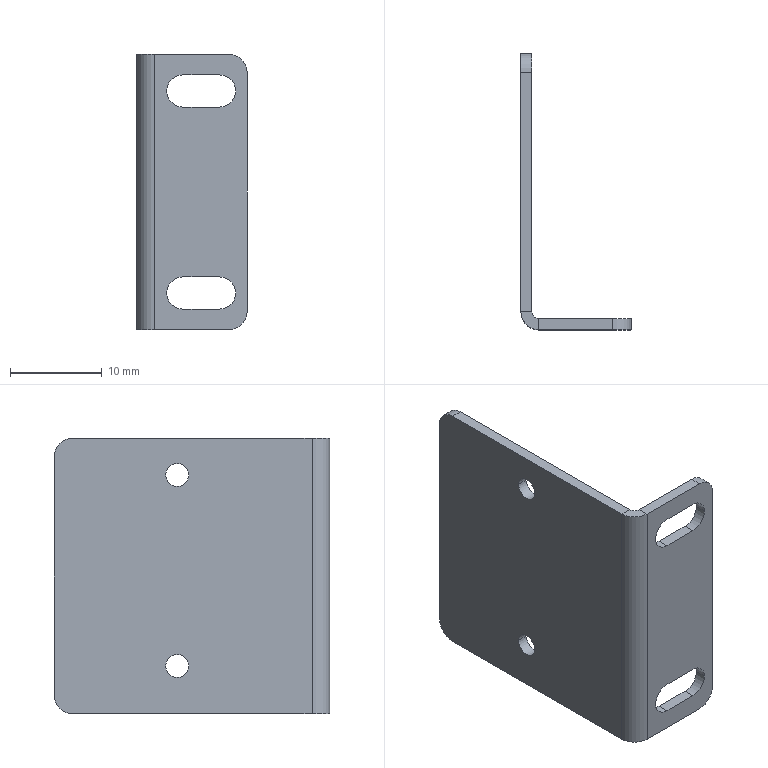Component | SolidWorks | SensorPlate7-1 | 1 solid | 32 faces | box 12 x 30 x 30 mm | volume 1376 mm3 | cylinder 16 | plane 16 | commonest cylinder face diameters 3.5 x6 2.5 x4 4 x4 3.873 x1 1.473 x1
STEP:
#1=COLOUR_RGB('',0.7922,0.8196,0.9333);
#2=FILL_AREA_STYLE_COLOUR('',#1);
#3=FILL_AREA_STYLE('',(#2));
#4=SURFACE_STYLE_FILL_AREA(#3);
#5=SURFACE_SIDE_STYLE('',(#4));
#6=SURFACE_STYLE_USAGE(.BOTH.,#5);
#7=PRESENTATION_STYLE_ASSIGNMENT((#6));
#8=CARTESIAN_POINT('',(-0.927,2.714,-3.325));
#9=VERTEX_POINT('',#8);
#10=CARTESIAN_POINT('',(-0.9958,2.714,-3.394));
#11=VERTEX_POINT('',#10);
#12=CARTESIAN_POINT('',(-0.9958,2.714,-3.325));
#13=DIRECTION('',(0.,1.,0.));
#14=DIRECTION('',(-1.,0.,0.));
#15=AXIS2_PLACEMENT_3D('',#12,#13,#14);
#16=CIRCLE('',#15,0.0689);
#17=EDGE_CURVE('',#9,#11,#16,.T.);
#18=ORIENTED_EDGE('',*,*,#17,.F.);
#19=CARTESIAN_POINT('',(-0.927,2.762,-3.325));
#20=VERTEX_POINT('',#19);
#21=CARTESIAN_POINT('',(-0.927,2.368,-3.325));
#22=DIRECTION('',(0.,1.,0.));
#23=VECTOR('',#22,39.37);
#24=LINE('',#21,#23);
#25=EDGE_CURVE('',#9,#20,#24,.T.);
#26=ORIENTED_EDGE('',*,*,#25,.T.);
#27=CARTESIAN_POINT('',(-0.9958,2.762,-3.394));
#28=VERTEX_POINT('',#27);
#29=CARTESIAN_POINT('',(-0.9958,2.762,-3.325));
#30=DIRECTION('',(-0.,-1.,-0.));
#31=DIRECTION('',(-1.,0.,0.));
#32=AXIS2_PLACEMENT_3D('',#29,#30,#31);
#33=CIRCLE('',#32,0.0689);
#34=EDGE_CURVE('',#28,#20,#33,.T.);
#35=ORIENTED_EDGE('',*,*,#34,.F.);
#36=CARTESIAN_POINT('',(-0.9958,2.368,-3.394));
#37=DIRECTION('',(0.,1.,0.));
#38=VECTOR('',#37,39.37);
#39=LINE('',#36,#38);
#40=EDGE_CURVE('',#11,#28,#39,.T.);
#41=ORIENTED_EDGE('',*,*,#40,.F.);
#42=EDGE_LOOP('',(#18,#26,#35,#41));
#43=FACE_OUTER_BOUND('',#42,.T.);
#44=CARTESIAN_POINT('',(-0.9958,2.368,-3.325));
#45=DIRECTION('',(0.,1.,0.));
#46=DIRECTION('',(1.,0.,0.));
#47=AXIS2_PLACEMENT_3D('',#44,#45,#46);
#48=CYLINDRICAL_SURFACE('',#47,0.0689);
#49=ADVANCED_FACE('',(#43),#48,.F.);
#50=CARTESIAN_POINT('',(-0.9958,2.714,-4.26));
#51=VERTEX_POINT('',#50);
#52=CARTESIAN_POINT('',(-0.927,2.714,-4.191));
#53=VERTEX_POINT('',#52);
#54=CARTESIAN_POINT('',(-0.9958,2.714,-4.191));
#55=DIRECTION('',(-0.,-1.,-0.));
#56=DIRECTION('',(-1.,0.,0.));
#57=AXIS2_PLACEMENT_3D('',#54,#55,#56);
#58=CIRCLE('',#57,0.0689);
#59=EDGE_CURVE('',#51,#53,#58,.T.);
#60=ORIENTED_EDGE('',*,*,#59,.T.);
#61=CARTESIAN_POINT('',(-0.927,2.762,-4.191));
#62=VERTEX_POINT('',#61);
#63=CARTESIAN_POINT('',(-0.927,2.368,-4.191));
#64=DIRECTION('',(0.,1.,0.));
#65=VECTOR('',#64,39.37);
#66=LINE('',#63,#65);
#67=EDGE_CURVE('',#53,#62,#66,.T.);
#68=ORIENTED_EDGE('',*,*,#67,.T.);
#69=CARTESIAN_POINT('',(-0.9958,2.762,-4.26));
#70=VERTEX_POINT('',#69);
#71=CARTESIAN_POINT('',(-0.9958,2.762,-4.191));
#72=DIRECTION('',(0.,1.,0.));
#73=DIRECTION('',(1.,0.,0.));
#74=AXIS2_PLACEMENT_3D('',#71,#72,#73);
#75=CIRCLE('',#74,0.0689);
#76=EDGE_CURVE('',#62,#70,#75,.T.);
#77=ORIENTED_EDGE('',*,*,#76,.T.);
#78=CARTESIAN_POINT('',(-0.9958,2.368,-4.26));
#79=DIRECTION('',(0.,1.,0.));
#80=VECTOR('',#79,39.37);
#81=LINE('',#78,#80);
#82=EDGE_CURVE('',#51,#70,#81,.T.);
#83=ORIENTED_EDGE('',*,*,#82,.F.);
#84=EDGE_LOOP('',(#60,#68,#77,#83));
#85=FACE_OUTER_BOUND('',#84,.T.);
#86=CARTESIAN_POINT('',(-0.9958,2.368,-4.191));
#87=DIRECTION('',(0.,1.,0.));
#88=DIRECTION('',(1.,0.,0.));
#89=AXIS2_PLACEMENT_3D('',#86,#87,#88);
#90=CYLINDRICAL_SURFACE('',#89,0.0689);
#91=ADVANCED_FACE('',(#85),#90,.F.);
#92=CARTESIAN_POINT('',(-1.303,3.417,-4.144));
#93=VERTEX_POINT('',#92);
#94=CARTESIAN_POINT('',(-1.303,3.319,-4.144));
#95=VERTEX_POINT('',#94);
#96=CARTESIAN_POINT('',(-1.303,3.368,-4.144));
#97=DIRECTION('',(1.,0.,-0.));
#98=DIRECTION('',(0.,-1.,0.));
#99=AXIS2_PLACEMENT_3D('',#96,#97,#98);
#100=CIRCLE('',#99,0.04921);
#101=EDGE_CURVE('',#93,#95,#100,.T.);
#102=ORIENTED_EDGE('',*,*,#101,.T.);
#103=CARTESIAN_POINT('',(-1.35,3.319,-4.144));
#104=VERTEX_POINT('',#103);
#105=CARTESIAN_POINT('',(-1.35,3.319,-4.144));
#106=DIRECTION('',(-1.,-0.,0.));
#107=VECTOR('',#106,39.37);
#108=LINE('',#105,#107);
#109=EDGE_CURVE('',#95,#104,#108,.T.);
#110=ORIENTED_EDGE('',*,*,#109,.T.);
#111=CARTESIAN_POINT('',(-1.35,3.417,-4.144));
#112=VERTEX_POINT('',#111);
#113=CARTESIAN_POINT('',(-1.35,3.368,-4.144));
#114=DIRECTION('',(-1.,-0.,0.));
#115=DIRECTION('',(0.,1.,0.));
#116=AXIS2_PLACEMENT_3D('',#113,#114,#115);
#117=CIRCLE('',#116,0.04921);
#118=EDGE_CURVE('',#104,#112,#117,.T.);
#119=ORIENTED_EDGE('',*,*,#118,.T.);
#120=CARTESIAN_POINT('',(-1.35,3.417,-4.144));
#121=DIRECTION('',(-1.,-0.,0.));
#122=VECTOR('',#121,39.37);
#123=LINE('',#120,#122);
#124=EDGE_CURVE('',#93,#112,#123,.T.);
#125=ORIENTED_EDGE('',*,*,#124,.F.);
#126=EDGE_LOOP('',(#102,#110,#119,#125));
#127=FACE_OUTER_BOUND('',#126,.T.);
#128=CARTESIAN_POINT('',(-1.35,3.368,-4.144));
#129=DIRECTION('',(-1.,-0.,0.));
#130=DIRECTION('',(0.,1.,0.));
#131=AXIS2_PLACEMENT_3D('',#128,#129,#130);
#132=CYLINDRICAL_SURFACE('',#131,0.04921);
#133=ADVANCED_FACE('',(#127),#132,.F.);
#134=CARTESIAN_POINT('',(-1.303,3.417,-3.325));
#135=VERTEX_POINT('',#134);
#136=CARTESIAN_POINT('',(-1.303,3.319,-3.325));
#137=VERTEX_POINT('',#136);
#138=CARTESIAN_POINT('',(-1.303,3.368,-3.325));
#139=DIRECTION('',(1.,0.,-0.));
#140=DIRECTION('',(0.,-1.,0.));
#141=AXIS2_PLACEMENT_3D('',#138,#139,#140);
#142=CIRCLE('',#141,0.04921);
#143=EDGE_CURVE('',#135,#137,#142,.T.);
#144=ORIENTED_EDGE('',*,*,#143,.T.);
#145=CARTESIAN_POINT('',(-1.35,3.319,-3.325));
#146=VERTEX_POINT('',#145);
#147=CARTESIAN_POINT('',(-1.35,3.319,-3.325));
#148=DIRECTION('',(-1.,-0.,0.));
#149=VECTOR('',#148,39.37);
#150=LINE('',#147,#149);
#151=EDGE_CURVE('',#137,#146,#150,.T.);
#152=ORIENTED_EDGE('',*,*,#151,.T.);
#153=CARTESIAN_POINT('',(-1.35,3.417,-3.325));
#154=VERTEX_POINT('',#153);
#155=CARTESIAN_POINT('',(-1.35,3.368,-3.325));
#156=DIRECTION('',(-1.,-0.,0.));
#157=DIRECTION('',(0.,1.,0.));
#158=AXIS2_PLACEMENT_3D('',#155,#156,#157);
#159=CIRCLE('',#158,0.04921);
#160=EDGE_CURVE('',#146,#154,#159,.T.);
#161=ORIENTED_EDGE('',*,*,#160,.T.);
#162=CARTESIAN_POINT('',(-1.35,3.417,-3.325));
#163=DIRECTION('',(-1.,-0.,0.));
#164=VECTOR('',#163,39.37);
#165=LINE('',#162,#164);
#166=EDGE_CURVE('',#135,#154,#165,.T.);
#167=ORIENTED_EDGE('',*,*,#166,.F.);
#168=EDGE_LOOP('',(#144,#152,#161,#167));
#169=FACE_OUTER_BOUND('',#168,.T.);
#170=CARTESIAN_POINT('',(-1.35,3.368,-3.325));
#171=DIRECTION('',(-1.,-0.,0.));
#172=DIRECTION('',(0.,1.,0.));
#173=AXIS2_PLACEMENT_3D('',#170,#171,#172);
#174=CYLINDRICAL_SURFACE('',#173,0.04921);
#175=ADVANCED_FACE('',(#169),#174,.F.);
#176=ORIENTED_EDGE('',*,*,#59,.F.);
#177=CARTESIAN_POINT('',(-1.153,2.714,-4.26));
#178=VERTEX_POINT('',#177);
#179=CARTESIAN_POINT('',(-1.303,2.714,-4.26));
#180=DIRECTION('',(1.,-0.,0.));
#181=VECTOR('',#180,39.37);
#182=LINE('',#179,#181);
#183=EDGE_CURVE('',#178,#51,#182,.T.);
#184=ORIENTED_EDGE('',*,*,#183,.F.);
#185=CARTESIAN_POINT('',(-1.153,2.714,-4.122));
#186=VERTEX_POINT('',#185);
#187=CARTESIAN_POINT('',(-1.153,2.714,-4.191));
#188=DIRECTION('',(-0.,-1.,-0.));
#189=DIRECTION('',(-1.,0.,0.));
#190=AXIS2_PLACEMENT_3D('',#187,#188,#189);
#191=CIRCLE('',#190,0.0689);
#192=EDGE_CURVE('',#186,#178,#191,.T.);
#193=ORIENTED_EDGE('',*,*,#192,.F.);
#194=CARTESIAN_POINT('',(-0.9958,2.714,-4.122));
#195=VERTEX_POINT('',#194);
#196=CARTESIAN_POINT('',(-1.303,2.714,-4.122));
#197=DIRECTION('',(1.,-0.,-0.));
#198=VECTOR('',#197,39.37);
#199=LINE('',#196,#198);
#200=EDGE_CURVE('',#186,#195,#199,.T.);
#201=ORIENTED_EDGE('',*,*,#200,.T.);
#202=CARTESIAN_POINT('',(-0.9958,2.714,-4.191));
#203=DIRECTION('',(-0.,-1.,-0.));
#204=DIRECTION('',(-1.,0.,0.));
#205=AXIS2_PLACEMENT_3D('',#202,#203,#204);
#206=CIRCLE('',#205,0.0689);
#207=EDGE_CURVE('',#53,#195,#206,.T.);
#208=ORIENTED_EDGE('',*,*,#207,.F.);
#209=EDGE_LOOP('',(#176,#184,#193,#201,#208));
#210=FACE_BOUND('',#209,.T.);
#211=CARTESIAN_POINT('',(-0.9565,2.714,-4.348));
#212=VERTEX_POINT('',#211);
#213=CARTESIAN_POINT('',(-1.274,2.714,-4.348));
#214=VERTEX_POINT('',#213);
#215=CARTESIAN_POINT('',(-1.303,2.714,-4.348));
#216=DIRECTION('',(-1.,0.,0.));
#217=VECTOR('',#216,39.37);
#218=LINE('',#215,#217);
#219=EDGE_CURVE('',#212,#214,#218,.T.);
#220=ORIENTED_EDGE('',*,*,#219,.F.);
#221=CARTESIAN_POINT('',(-0.8777,2.714,-4.27));
#222=VERTEX_POINT('',#221);
#223=CARTESIAN_POINT('',(-0.9565,2.714,-4.27));
#224=DIRECTION('',(-0.,-1.,-0.));
#225=DIRECTION('',(-1.,0.,0.));
#226=AXIS2_PLACEMENT_3D('',#223,#224,#225);
#227=CIRCLE('',#226,0.07874);
#228=EDGE_CURVE('',#212,#222,#227,.T.);
#229=ORIENTED_EDGE('',*,*,#228,.T.);
#230=CARTESIAN_POINT('',(-0.8777,2.714,-3.246));
#231=VERTEX_POINT('',#230);
#232=CARTESIAN_POINT('',(-0.8777,2.714,-4.348));
#233=DIRECTION('',(-0.,0.,-1.));
#234=VECTOR('',#233,39.37);
#235=LINE('',#232,#234);
#236=EDGE_CURVE('',#231,#222,#235,.T.);
#237=ORIENTED_EDGE('',*,*,#236,.F.);
#238=CARTESIAN_POINT('',(-0.9565,2.714,-3.167));
#239=VERTEX_POINT('',#238);
#240=CARTESIAN_POINT('',(-0.9565,2.714,-3.246));
#241=DIRECTION('',(-0.,-1.,-0.));
#242=DIRECTION('',(-1.,0.,0.));
#243=AXIS2_PLACEMENT_3D('',#240,#241,#242);
#244=CIRCLE('',#243,0.07874);
#245=EDGE_CURVE('',#231,#239,#244,.T.);
#246=ORIENTED_EDGE('',*,*,#245,.T.);
#247=CARTESIAN_POINT('',(-1.274,2.714,-3.167));
#248=VERTEX_POINT('',#247);
#249=CARTESIAN_POINT('',(-0.8777,2.714,-3.167));
#250=DIRECTION('',(1.,-0.,-0.));
#251=VECTOR('',#250,39.37);
#252=LINE('',#249,#251);
#253=EDGE_CURVE('',#248,#239,#252,.T.);
#254=ORIENTED_EDGE('',*,*,#253,.F.);
#255=CARTESIAN_POINT('',(-1.274,2.714,-3.561));
#256=DIRECTION('',(-0.,0.,-1.));
#257=VECTOR('',#256,39.37);
#258=LINE('',#255,#257);
#259=EDGE_CURVE('',#248,#214,#258,.T.);
#260=ORIENTED_EDGE('',*,*,#259,.T.);
#261=EDGE_LOOP('',(#220,#229,#237,#246,#254,#260));
#262=FACE_OUTER_BOUND('',#261,.T.);
#263=CARTESIAN_POINT('',(-1.153,2.714,-3.256));
#264=VERTEX_POINT('',#263);
#265=CARTESIAN_POINT('',(-0.9958,2.714,-3.256));
#266=VERTEX_POINT('',#265);
#267=CARTESIAN_POINT('',(-1.303,2.714,-3.256));
#268=DIRECTION('',(1.,-0.,-0.));
#269=VECTOR('',#268,39.37);
#270=LINE('',#267,#269);
#271=EDGE_CURVE('',#264,#266,#270,.T.);
#272=ORIENTED_EDGE('',*,*,#271,.T.);
#273=CARTESIAN_POINT('',(-0.9958,2.714,-3.325));
#274=DIRECTION('',(0.,1.,0.));
#275=DIRECTION('',(-1.,0.,0.));
#276=AXIS2_PLACEMENT_3D('',#273,#274,#275);
#277=CIRCLE('',#276,0.0689);
#278=EDGE_CURVE('',#266,#9,#277,.T.);
#279=ORIENTED_EDGE('',*,*,#278,.T.);
#280=ORIENTED_EDGE('',*,*,#17,.T.);
#281=CARTESIAN_POINT('',(-1.153,2.714,-3.394));
#282=VERTEX_POINT('',#281);
#283=CARTESIAN_POINT('',(-1.303,2.714,-3.394));
#284=DIRECTION('',(1.,-0.,-0.));
#285=VECTOR('',#284,39.37);
#286=LINE('',#283,#285);
#287=EDGE_CURVE('',#282,#11,#286,.T.);
#288=ORIENTED_EDGE('',*,*,#287,.F.);
#289=CARTESIAN_POINT('',(-1.153,2.714,-3.325));
#290=DIRECTION('',(0.,1.,0.));
#291=DIRECTION('',(-1.,0.,0.));
#292=AXIS2_PLACEMENT_3D('',#289,#290,#291);
#293=CIRCLE('',#292,0.0689);
#294=EDGE_CURVE('',#282,#264,#293,.T.);
#295=ORIENTED_EDGE('',*,*,#294,.T.);
#296=EDGE_LOOP('',(#272,#279,#280,#288,#295));
#297=FACE_BOUND('',#296,.T.);
#298=CARTESIAN_POINT('',(-1.303,2.714,-3.561));
#299=DIRECTION('',(-0.,-1.,-0.));
#300=DIRECTION('',(-1.,0.,0.));
#301=AXIS2_PLACEMENT_3D('',#298,#299,#300);
#302=PLANE('',#301);
#303=ADVANCED_FACE('',(#210,#262,#297),#302,.T.);
#304=CARTESIAN_POINT('',(-0.8777,2.762,-3.246));
#305=VERTEX_POINT('',#304);
#306=CARTESIAN_POINT('',(-0.8777,2.762,-4.27));
#307=VERTEX_POINT('',#306);
#308=CARTESIAN_POINT('',(-0.8777,2.762,-3.561));
#309=DIRECTION('',(-0.,0.,-1.));
#310=VECTOR('',#309,39.37);
#311=LINE('',#308,#310);
#312=EDGE_CURVE('',#305,#307,#311,.T.);
#313=ORIENTED_EDGE('',*,*,#312,.T.);
#314=CARTESIAN_POINT('',(-0.9565,2.762,-4.348));
#315=VERTEX_POINT('',#314);
#316=CARTESIAN_POINT('',(-0.9565,2.762,-4.27));
#317=DIRECTION('',(0.,1.,0.));
#318=DIRECTION('',(-1.,0.,0.));
#319=AXIS2_PLACEMENT_3D('',#316,#317,#318);
#320=CIRCLE('',#319,0.07874);
#321=EDGE_CURVE('',#307,#315,#320,.T.);
#322=ORIENTED_EDGE('',*,*,#321,.T.);
#323=CARTESIAN_POINT('',(-1.274,2.762,-4.348));
#324=VERTEX_POINT('',#323);
#325=CARTESIAN_POINT('',(-1.303,2.762,-4.348));
#326=DIRECTION('',(-1.,0.,0.));
#327=VECTOR('',#326,39.37);
#328=LINE('',#325,#327);
#329=EDGE_CURVE('',#315,#324,#328,.T.);
#330=ORIENTED_EDGE('',*,*,#329,.T.);
#331=CARTESIAN_POINT('',(-1.274,2.762,-3.167));
#332=VERTEX_POINT('',#331);
#333=CARTESIAN_POINT('',(-1.274,2.762,-3.167));
#334=DIRECTION('',(-0.,0.,-1.));
#335=VECTOR('',#334,39.37);
#336=LINE('',#333,#335);
#337=EDGE_CURVE('',#332,#324,#336,.T.);
#338=ORIENTED_EDGE('',*,*,#337,.F.);
#339=CARTESIAN_POINT('',(-0.9565,2.762,-3.167));
#340=VERTEX_POINT('',#339);
#341=CARTESIAN_POINT('',(-1.303,2.762,-3.167));
#342=DIRECTION('',(1.,-0.,-0.));
#343=VECTOR('',#342,39.37);
#344=LINE('',#341,#343);
#345=EDGE_CURVE('',#332,#340,#344,.T.);
#346=ORIENTED_EDGE('',*,*,#345,.T.);
#347=CARTESIAN_POINT('',(-0.9565,2.762,-3.246));
#348=DIRECTION('',(0.,1.,0.));
#349=DIRECTION('',(-1.,0.,0.));
#350=AXIS2_PLACEMENT_3D('',#347,#348,#349);
#351=CIRCLE('',#350,0.07874);
#352=EDGE_CURVE('',#340,#305,#351,.T.);
#353=ORIENTED_EDGE('',*,*,#352,.T.);
#354=EDGE_LOOP('',(#313,#322,#330,#338,#346,#353));
#355=FACE_OUTER_BOUND('',#354,.T.);
#356=CARTESIAN_POINT('',(-1.153,2.762,-4.26));
#357=VERTEX_POINT('',#356);
#358=CARTESIAN_POINT('',(-0.9958,2.762,-4.26));
#359=DIRECTION('',(-1.,0.,-0.));
#360=VECTOR('',#359,39.37);
#361=LINE('',#358,#360);
#362=EDGE_CURVE('',#70,#357,#361,.T.);
#363=ORIENTED_EDGE('',*,*,#362,.F.);
#364=ORIENTED_EDGE('',*,*,#76,.F.);
#365=CARTESIAN_POINT('',(-0.9958,2.762,-4.122));
#366=VERTEX_POINT('',#365);
#367=CARTESIAN_POINT('',(-0.9958,2.762,-4.191));
#368=DIRECTION('',(0.,1.,0.));
#369=DIRECTION('',(1.,0.,0.));
#370=AXIS2_PLACEMENT_3D('',#367,#368,#369);
#371=CIRCLE('',#370,0.0689);
#372=EDGE_CURVE('',#366,#62,#371,.T.);
#373=ORIENTED_EDGE('',*,*,#372,.F.);
#374=CARTESIAN_POINT('',(-1.153,2.762,-4.122));
#375=VERTEX_POINT('',#374);
#376=CARTESIAN_POINT('',(-0.9958,2.762,-4.122));
#377=DIRECTION('',(-1.,0.,0.));
#378=VECTOR('',#377,39.37);
#379=LINE('',#376,#378);
#380=EDGE_CURVE('',#366,#375,#379,.T.);
#381=ORIENTED_EDGE('',*,*,#380,.T.);
#382=CARTESIAN_POINT('',(-1.153,2.762,-4.191));
#383=DIRECTION('',(0.,1.,0.));
#384=DIRECTION('',(1.,0.,0.));
#385=AXIS2_PLACEMENT_3D('',#382,#383,#384);
#386=CIRCLE('',#385,0.0689);
#387=EDGE_CURVE('',#357,#375,#386,.T.);
#388=ORIENTED_EDGE('',*,*,#387,.F.);
#389=EDGE_LOOP('',(#363,#364,#373,#381,#388));
#390=FACE_BOUND('',#389,.T.);
#391=ORIENTED_EDGE('',*,*,#34,.T.);
#392=CARTESIAN_POINT('',(-0.9958,2.762,-3.256));
#393=VERTEX_POINT('',#392);
#394=CARTESIAN_POINT('',(-0.9958,2.762,-3.325));
#395=DIRECTION('',(-0.,-1.,-0.));
#396=DIRECTION('',(-1.,0.,0.));
#397=AXIS2_PLACEMENT_3D('',#394,#395,#396);
#398=CIRCLE('',#397,0.0689);
#399=EDGE_CURVE('',#20,#393,#398,.T.);
#400=ORIENTED_EDGE('',*,*,#399,.T.);
#401=CARTESIAN_POINT('',(-1.153,2.762,-3.256));
#402=VERTEX_POINT('',#401);
#403=CARTESIAN_POINT('',(-0.9958,2.762,-3.256));
#404=DIRECTION('',(-1.,0.,0.));
#405=VECTOR('',#404,39.37);
#406=LINE('',#403,#405);
#407=EDGE_CURVE('',#393,#402,#406,.T.);
#408=ORIENTED_EDGE('',*,*,#407,.T.);
#409=CARTESIAN_POINT('',(-1.153,2.762,-3.394));
#410=VERTEX_POINT('',#409);
#411=CARTESIAN_POINT('',(-1.153,2.762,-3.325));
#412=DIRECTION('',(-0.,-1.,-0.));
#413=DIRECTION('',(-1.,0.,0.));
#414=AXIS2_PLACEMENT_3D('',#411,#412,#413);
#415=CIRCLE('',#414,0.0689);
#416=EDGE_CURVE('',#402,#410,#415,.T.);
#417=ORIENTED_EDGE('',*,*,#416,.T.);
#418=CARTESIAN_POINT('',(-0.9958,2.762,-3.394));
#419=DIRECTION('',(-1.,0.,0.));
#420=VECTOR('',#419,39.37);
#421=LINE('',#418,#420);
#422=EDGE_CURVE('',#28,#410,#421,.T.);
#423=ORIENTED_EDGE('',*,*,#422,.F.);
#424=EDGE_LOOP('',(#391,#400,#408,#417,#423));
#425=FACE_BOUND('',#424,.T.);
#426=CARTESIAN_POINT('',(-1.303,2.762,-3.561));
#427=DIRECTION('',(-0.,-1.,-0.));
#428=DIRECTION('',(-1.,0.,0.));
#429=AXIS2_PLACEMENT_3D('',#426,#427,#428);
#430=PLANE('',#429);
#431=ADVANCED_FACE('',(#355,#390,#425),#430,.F.);
#432=CARTESIAN_POINT('',(-1.35,3.368,-4.144));
#433=DIRECTION('',(-1.,-0.,0.));
#434=DIRECTION('',(0.,1.,0.));
#435=AXIS2_PLACEMENT_3D('',#432,#433,#434);
#436=CIRCLE('',#435,0.04921);
#437=EDGE_CURVE('',#112,#104,#436,.T.);
#438=ORIENTED_EDGE('',*,*,#437,.F.);
#439=ORIENTED_EDGE('',*,*,#118,.F.);
#440=EDGE_LOOP('',(#438,#439));
#441=FACE_BOUND('',#440,.T.);
#442=CARTESIAN_POINT('',(-1.35,3.368,-3.325));
#443=DIRECTION('',(-1.,-0.,0.));
#444=DIRECTION('',(0.,1.,0.));
#445=AXIS2_PLACEMENT_3D('',#442,#443,#444);
#446=CIRCLE('',#445,0.04921);
#447=EDGE_CURVE('',#154,#146,#446,.T.);
#448=ORIENTED_EDGE('',*,*,#447,.F.);
#449=ORIENTED_EDGE('',*,*,#160,.F.);
#450=EDGE_LOOP('',(#448,#449));
#451=FACE_BOUND('',#450,.T.);
#452=CARTESIAN_POINT('',(-1.35,3.895,-3.246));
#453=VERTEX_POINT('',#452);
#454=CARTESIAN_POINT('',(-1.35,3.895,-4.27));
#455=VERTEX_POINT('',#454);
#456=CARTESIAN_POINT('',(-1.35,3.895,-3.167));
#457=DIRECTION('',(-0.,0.,-1.));
#458=VECTOR('',#457,39.37);
#459=LINE('',#456,#458);
#460=EDGE_CURVE('',#453,#455,#459,.T.);
#461=ORIENTED_EDGE('',*,*,#460,.T.);
#462=CARTESIAN_POINT('',(-1.35,3.817,-4.348));
#463=VERTEX_POINT('',#462);
#464=CARTESIAN_POINT('',(-1.35,3.817,-4.27));
#465=DIRECTION('',(-1.,-0.,0.));
#466=DIRECTION('',(0.,-1.,0.));
#467=AXIS2_PLACEMENT_3D('',#464,#465,#466);
#468=CIRCLE('',#467,0.07874);
#469=EDGE_CURVE('',#455,#463,#468,.T.);
#470=ORIENTED_EDGE('',*,*,#469,.T.);
#471=CARTESIAN_POINT('',(-1.35,2.791,-4.348));
#472=VERTEX_POINT('',#471);
#473=CARTESIAN_POINT('',(-1.35,2.714,-4.348));
#474=DIRECTION('',(-0.,1.,0.));
#475=VECTOR('',#474,39.37);
#476=LINE('',#473,#475);
#477=EDGE_CURVE('',#472,#463,#476,.T.);
#478=ORIENTED_EDGE('',*,*,#477,.F.);
#479=CARTESIAN_POINT('',(-1.35,2.791,-3.167));
#480=VERTEX_POINT('',#479);
#481=CARTESIAN_POINT('',(-1.35,2.791,-4.348));
#482=DIRECTION('',(0.,-0.,1.));
#483=VECTOR('',#482,39.37);
#484=LINE('',#481,#483);
#485=EDGE_CURVE('',#472,#480,#484,.T.);
#486=ORIENTED_EDGE('',*,*,#485,.T.);
#487=CARTESIAN_POINT('',(-1.35,3.817,-3.167));
#488=VERTEX_POINT('',#487);
#489=CARTESIAN_POINT('',(-1.35,2.714,-3.167));
#490=DIRECTION('',(-0.,1.,0.));
#491=VECTOR('',#490,39.37);
#492=LINE('',#489,#491);
#493=EDGE_CURVE('',#480,#488,#492,.T.);
#494=ORIENTED_EDGE('',*,*,#493,.T.);
#495=CARTESIAN_POINT('',(-1.35,3.817,-3.246));
#496=DIRECTION('',(-1.,-0.,0.));
#497=DIRECTION('',(0.,-1.,0.));
#498=AXIS2_PLACEMENT_3D('',#495,#496,#497);
#499=CIRCLE('',#498,0.07874);
#500=EDGE_CURVE('',#488,#453,#499,.T.);
#501=ORIENTED_EDGE('',*,*,#500,.T.);
#502=EDGE_LOOP('',(#461,#470,#478,#486,#494,#501));
#503=FACE_OUTER_BOUND('',#502,.T.);
#504=CARTESIAN_POINT('',(-1.35,2.714,-3.167));
#505=DIRECTION('',(1.,0.,-0.));
#506=DIRECTION('',(0.,-1.,-0.));
#507=AXIS2_PLACEMENT_3D('',#504,#505,#506);
#508=PLANE('',#507);
#509=ADVANCED_FACE('',(#441,#451,#503),#508,.F.);
#510=ORIENTED_EDGE('',*,*,#477,.T.);
#511=CARTESIAN_POINT('',(-1.303,3.817,-4.348));
#512=VERTEX_POINT('',#511);
#513=CARTESIAN_POINT('',(-1.303,3.817,-4.348));
#514=DIRECTION('',(1.,0.,-0.));
#515=VECTOR('',#514,39.37);
#516=LINE('',#513,#515);
#517=EDGE_CURVE('',#463,#512,#516,.T.);
#518=ORIENTED_EDGE('',*,*,#517,.T.);
#519=CARTESIAN_POINT('',(-1.303,2.791,-4.348));
#520=VERTEX_POINT('',#519);
#521=CARTESIAN_POINT('',(-1.303,2.714,-4.348));
#522=DIRECTION('',(-0.,1.,0.));
#523=VECTOR('',#522,39.37);
#524=LINE('',#521,#523);
#525=EDGE_CURVE('',#520,#512,#524,.T.);
#526=ORIENTED_EDGE('',*,*,#525,.F.);
#527=CARTESIAN_POINT('',(-1.303,2.791,-4.348));
#528=DIRECTION('',(-1.,-0.,0.));
#529=VECTOR('',#528,39.37);
#530=LINE('',#527,#529);
#531=EDGE_CURVE('',#520,#472,#530,.T.);
#532=ORIENTED_EDGE('',*,*,#531,.T.);
#533=EDGE_LOOP('',(#510,#518,#526,#532));
#534=FACE_OUTER_BOUND('',#533,.T.);
#535=CARTESIAN_POINT('',(-1.303,2.714,-4.348));
#536=DIRECTION('',(-0.,0.,-1.));
#537=DIRECTION('',(-0.,1.,0.));
#538=AXIS2_PLACEMENT_3D('',#535,#536,#537);
#539=PLANE('',#538);
#540=ADVANCED_FACE('',(#534),#539,.T.);
#541=ORIENTED_EDGE('',*,*,#101,.F.);
#542=CARTESIAN_POINT('',(-1.303,3.368,-4.144));
#543=DIRECTION('',(1.,0.,-0.));
#544=DIRECTION('',(0.,-1.,0.));
#545=AXIS2_PLACEMENT_3D('',#542,#543,#544);
#546=CIRCLE('',#545,0.04921);
#547=EDGE_CURVE('',#95,#93,#546,.T.);
#548=ORIENTED_EDGE('',*,*,#547,.F.);
#549=EDGE_LOOP('',(#541,#548));
#550=FACE_BOUND('',#549,.T.);
#551=ORIENTED_EDGE('',*,*,#143,.F.);
#552=CARTESIAN_POINT('',(-1.303,3.368,-3.325));
#553=DIRECTION('',(1.,0.,-0.));
#554=DIRECTION('',(0.,-1.,0.));
#555=AXIS2_PLACEMENT_3D('',#552,#553,#554);
#556=CIRCLE('',#555,0.04921);
#557=EDGE_CURVE('',#137,#135,#556,.T.);
#558=ORIENTED_EDGE('',*,*,#557,.F.);
#559=EDGE_LOOP('',(#551,#558));
#560=FACE_BOUND('',#559,.T.);
#561=ORIENTED_EDGE('',*,*,#525,.T.);
#562=CARTESIAN_POINT('',(-1.303,3.895,-4.27));
#563=VERTEX_POINT('',#562);
#564=CARTESIAN_POINT('',(-1.303,3.817,-4.27));
#565=DIRECTION('',(1.,0.,-0.));
#566=DIRECTION('',(0.,-1.,0.));
#567=AXIS2_PLACEMENT_3D('',#564,#565,#566);
#568=CIRCLE('',#567,0.07874);
#569=EDGE_CURVE('',#512,#563,#568,.T.);
#570=ORIENTED_EDGE('',*,*,#569,.T.);
#571=CARTESIAN_POINT('',(-1.303,3.895,-3.246));
#572=VERTEX_POINT('',#571);
#573=CARTESIAN_POINT('',(-1.303,3.895,-3.167));
#574=DIRECTION('',(-0.,0.,-1.));
#575=VECTOR('',#574,39.37);
#576=LINE('',#573,#575);
#577=EDGE_CURVE('',#572,#563,#576,.T.);
#578=ORIENTED_EDGE('',*,*,#577,.F.);
#579=CARTESIAN_POINT('',(-1.303,3.817,-3.167));
#580=VERTEX_POINT('',#579);
#581=CARTESIAN_POINT('',(-1.303,3.817,-3.246));
#582=DIRECTION('',(1.,0.,-0.));
#583=DIRECTION('',(0.,-1.,0.));
#584=AXIS2_PLACEMENT_3D('',#581,#582,#583);
#585=CIRCLE('',#584,0.07874);
#586=EDGE_CURVE('',#572,#580,#585,.T.);
#587=ORIENTED_EDGE('',*,*,#586,.T.);
#588=CARTESIAN_POINT('',(-1.303,2.791,-3.167));
#589=VERTEX_POINT('',#588);
#590=CARTESIAN_POINT('',(-1.303,2.714,-3.167));
#591=DIRECTION('',(-0.,1.,0.));
#592=VECTOR('',#591,39.37);
#593=LINE('',#590,#592);
#594=EDGE_CURVE('',#589,#580,#593,.T.);
#595=ORIENTED_EDGE('',*,*,#594,.F.);
#596=CARTESIAN_POINT('',(-1.303,2.791,-4.348));
#597=DIRECTION('',(0.,-0.,1.));
#598=VECTOR('',#597,39.37);
#599=LINE('',#596,#598);
#600=EDGE_CURVE('',#520,#589,#599,.T.);
#601=ORIENTED_EDGE('',*,*,#600,.F.);
#602=EDGE_LOOP('',(#561,#570,#578,#587,#595,#601));
#603=FACE_OUTER_BOUND('',#602,.T.);
#604=CARTESIAN_POINT('',(-1.303,2.714,-3.167));
#605=DIRECTION('',(1.,0.,-0.));
#606=DIRECTION('',(0.,-1.,-0.));
#607=AXIS2_PLACEMENT_3D('',#604,#605,#606);
#608=PLANE('',#607);
#609=ADVANCED_FACE('',(#550,#560,#603),#608,.T.);
#610=ORIENTED_EDGE('',*,*,#594,.T.);
#611=CARTESIAN_POINT('',(-1.35,3.817,-3.167));
#612=DIRECTION('',(-1.,-0.,0.));
#613=VECTOR('',#612,39.37);
#614=LINE('',#611,#613);
#615=EDGE_CURVE('',#580,#488,#614,.T.);
#616=ORIENTED_EDGE('',*,*,#615,.T.);
#617=ORIENTED_EDGE('',*,*,#493,.F.);
#618=CARTESIAN_POINT('',(-1.303,2.791,-3.167));
#619=DIRECTION('',(-1.,-0.,0.));
#620=VECTOR('',#619,39.37);
#621=LINE('',#618,#620);
#622=EDGE_CURVE('',#589,#480,#621,.T.);
#623=ORIENTED_EDGE('',*,*,#622,.F.);
#624=EDGE_LOOP('',(#610,#616,#617,#623));
#625=FACE_OUTER_BOUND('',#624,.T.);
#626=CARTESIAN_POINT('',(-1.35,2.714,-3.167));
#627=DIRECTION('',(0.,-0.,1.));
#628=DIRECTION('',(0.,-1.,-0.));
#629=AXIS2_PLACEMENT_3D('',#626,#627,#628);
#630=PLANE('',#629);
#631=ADVANCED_FACE('',(#625),#630,.T.);
#632=ORIENTED_EDGE('',*,*,#577,.T.);
#633=CARTESIAN_POINT('',(-1.303,3.895,-4.27));
#634=DIRECTION('',(-1.,-0.,0.));
#635=VECTOR('',#634,39.37);
#636=LINE('',#633,#635);
#637=EDGE_CURVE('',#563,#455,#636,.T.);
#638=ORIENTED_EDGE('',*,*,#637,.T.);
#639=ORIENTED_EDGE('',*,*,#460,.F.);
#640=CARTESIAN_POINT('',(-1.303,3.895,-3.246));
#641=DIRECTION('',(1.,0.,-0.));
#642=VECTOR('',#641,39.37);
#643=LINE('',#640,#642);
#644=EDGE_CURVE('',#453,#572,#643,.T.);
#645=ORIENTED_EDGE('',*,*,#644,.T.);
#646=EDGE_LOOP('',(#632,#638,#639,#645));
#647=FACE_OUTER_BOUND('',#646,.T.);
#648=CARTESIAN_POINT('',(-1.303,3.895,-3.561));
#649=DIRECTION('',(-0.,1.,0.));
#650=DIRECTION('',(0.,-0.,1.));
#651=AXIS2_PLACEMENT_3D('',#648,#649,#650);
#652=PLANE('',#651);
#653=ADVANCED_FACE('',(#647),#652,.T.);
#654=CARTESIAN_POINT('',(-1.274,2.714,-3.167));
#655=DIRECTION('',(0.,-1.,-0.));
#656=VECTOR('',#655,39.37);
#657=LINE('',#654,#656);
#658=EDGE_CURVE('',#332,#248,#657,.T.);
#659=ORIENTED_EDGE('',*,*,#658,.F.);
#660=CARTESIAN_POINT('',(-1.274,2.791,-3.167));
#661=DIRECTION('',(0.,-0.,1.));
#662=DIRECTION('',(0.,1.,0.));
#663=AXIS2_PLACEMENT_3D('',#660,#661,#662);
#664=CIRCLE('',#663,0.029);
#665=EDGE_CURVE('',#589,#332,#664,.T.);
#666=ORIENTED_EDGE('',*,*,#665,.F.);
#667=ORIENTED_EDGE('',*,*,#622,.T.);
#668=CARTESIAN_POINT('',(-1.274,2.791,-3.167));
#669=DIRECTION('',(0.,-0.,1.));
#670=DIRECTION('',(-0.,1.,0.));
#671=AXIS2_PLACEMENT_3D('',#668,#669,#670);
#672=CIRCLE('',#671,0.07624);
#673=EDGE_CURVE('',#480,#248,#672,.T.);
#674=ORIENTED_EDGE('',*,*,#673,.T.);
#675=EDGE_LOOP('',(#659,#666,#667,#674));
#676=FACE_OUTER_BOUND('',#675,.T.);
#677=CARTESIAN_POINT('',(-1.274,2.791,-3.167));
#678=DIRECTION('',(0.,-0.,1.));
#679=DIRECTION('',(0.,-1.,-0.));
#680=AXIS2_PLACEMENT_3D('',#677,#678,#679);
#681=PLANE('',#680);
#682=ADVANCED_FACE('',(#676),#681,.T.);
#683=CARTESIAN_POINT('',(-1.274,2.791,-4.348));
#684=DIRECTION('',(-0.,0.,-1.));
#685=DIRECTION('',(0.,1.,0.));
#686=AXIS2_PLACEMENT_3D('',#683,#684,#685);
#687=CIRCLE('',#686,0.029);
#688=EDGE_CURVE('',#324,#520,#687,.T.);
#689=ORIENTED_EDGE('',*,*,#688,.F.);
#690=CARTESIAN_POINT('',(-1.274,2.762,-4.348));
#691=DIRECTION('',(0.,-1.,-0.));
#692=VECTOR('',#691,39.37);
#693=LINE('',#690,#692);
#694=EDGE_CURVE('',#324,#214,#693,.T.);
#695=ORIENTED_EDGE('',*,*,#694,.T.);
#696=CARTESIAN_POINT('',(-1.274,2.791,-4.348));
#697=DIRECTION('',(-0.,0.,-1.));
#698=DIRECTION('',(-0.,1.,0.));
#699=AXIS2_PLACEMENT_3D('',#696,#697,#698);
#700=CIRCLE('',#699,0.07624);
#701=EDGE_CURVE('',#214,#472,#700,.T.);
#702=ORIENTED_EDGE('',*,*,#701,.T.);
#703=ORIENTED_EDGE('',*,*,#531,.F.);
#704=EDGE_LOOP('',(#689,#695,#702,#703));
#705=FACE_OUTER_BOUND('',#704,.T.);
#706=CARTESIAN_POINT('',(-1.274,2.791,-4.348));
#707=DIRECTION('',(0.,-0.,1.));
#708=DIRECTION('',(0.,-1.,-0.));
#709=AXIS2_PLACEMENT_3D('',#706,#707,#708);
#710=PLANE('',#709);
#711=ADVANCED_FACE('',(#705),#710,.F.);
#712=ORIENTED_EDGE('',*,*,#485,.F.);
#713=ORIENTED_EDGE('',*,*,#701,.F.);
#714=ORIENTED_EDGE('',*,*,#259,.F.);
#715=ORIENTED_EDGE('',*,*,#673,.F.);
#716=EDGE_LOOP('',(#712,#713,#714,#715));
#717=FACE_OUTER_BOUND('',#716,.T.);
#718=CARTESIAN_POINT('',(-1.274,2.791,-4.348));
#719=DIRECTION('',(-0.,0.,-1.));
#720=DIRECTION('',(0.,-1.,0.));
#721=AXIS2_PLACEMENT_3D('',#718,#719,#720);
#722=CYLINDRICAL_SURFACE('',#721,0.07624);
#723=ADVANCED_FACE('',(#717),#722,.T.);
#724=ORIENTED_EDGE('',*,*,#600,.T.);
#725=ORIENTED_EDGE('',*,*,#665,.T.);
#726=ORIENTED_EDGE('',*,*,#337,.T.);
#727=ORIENTED_EDGE('',*,*,#688,.T.);
#728=EDGE_LOOP('',(#724,#725,#726,#727));
#729=FACE_OUTER_BOUND('',#728,.T.);
#730=CARTESIAN_POINT('',(-1.274,2.791,-4.348));
#731=DIRECTION('',(-0.,0.,-1.));
#732=DIRECTION('',(0.,-1.,0.));
#733=AXIS2_PLACEMENT_3D('',#730,#731,#732);
#734=CYLINDRICAL_SURFACE('',#733,0.029);
#735=ADVANCED_FACE('',(#729),#734,.F.);
#736=ORIENTED_EDGE('',*,*,#329,.F.);
#737=CARTESIAN_POINT('',(-0.9565,2.714,-4.348));
#738=DIRECTION('',(-0.,-1.,-0.));
#739=VECTOR('',#738,39.37);
#740=LINE('',#737,#739);
#741=EDGE_CURVE('',#315,#212,#740,.T.);
#742=ORIENTED_EDGE('',*,*,#741,.T.);
#743=ORIENTED_EDGE('',*,*,#219,.T.);
#744=ORIENTED_EDGE('',*,*,#694,.F.);
#745=EDGE_LOOP('',(#736,#742,#743,#744));
#746=FACE_OUTER_BOUND('',#745,.T.);
#747=CARTESIAN_POINT('',(-1.303,2.714,-4.348));
#748=DIRECTION('',(-0.,0.,-1.));
#749=DIRECTION('',(-0.,1.,0.));
#750=AXIS2_PLACEMENT_3D('',#747,#748,#749);
#751=PLANE('',#750);
#752=ADVANCED_FACE('',(#746),#751,.T.);
#753=ORIENTED_EDGE('',*,*,#253,.T.);
#754=CARTESIAN_POINT('',(-0.9565,2.714,-3.167));
#755=DIRECTION('',(0.,1.,0.));
#756=VECTOR('',#755,39.37);
#757=LINE('',#754,#756);
#758=EDGE_CURVE('',#239,#340,#757,.T.);
#759=ORIENTED_EDGE('',*,*,#758,.T.);
#760=ORIENTED_EDGE('',*,*,#345,.F.);
#761=ORIENTED_EDGE('',*,*,#658,.T.);
#762=EDGE_LOOP('',(#753,#759,#760,#761));
#763=FACE_OUTER_BOUND('',#762,.T.);
#764=CARTESIAN_POINT('',(-0.8777,2.714,-3.167));
#765=DIRECTION('',(0.,-0.,1.));
#766=DIRECTION('',(0.,-1.,-0.));
#767=AXIS2_PLACEMENT_3D('',#764,#765,#766);
#768=PLANE('',#767);
#769=ADVANCED_FACE('',(#763),#768,.T.);
#770=ORIENTED_EDGE('',*,*,#236,.T.);
#771=CARTESIAN_POINT('',(-0.8777,2.714,-4.27));
#772=DIRECTION('',(0.,1.,0.));
#773=VECTOR('',#772,39.37);
#774=LINE('',#771,#773);
#775=EDGE_CURVE('',#222,#307,#774,.T.);
#776=ORIENTED_EDGE('',*,*,#775,.T.);
#777=ORIENTED_EDGE('',*,*,#312,.F.);
#778=CARTESIAN_POINT('',(-0.8777,2.714,-3.246));
#779=DIRECTION('',(-0.,-1.,-0.));
#780=VECTOR('',#779,39.37);
#781=LINE('',#778,#780);
#782=EDGE_CURVE('',#305,#231,#781,.T.);
#783=ORIENTED_EDGE('',*,*,#782,.T.);
#784=EDGE_LOOP('',(#770,#776,#777,#783));
#785=FACE_OUTER_BOUND('',#784,.T.);
#786=CARTESIAN_POINT('',(-0.8777,2.714,-4.348));
#787=DIRECTION('',(1.,-0.,-0.));
#788=DIRECTION('',(-0.,-1.,-0.));
#789=AXIS2_PLACEMENT_3D('',#786,#787,#788);
#790=PLANE('',#789);
#791=ADVANCED_FACE('',(#785),#790,.T.);
#792=ORIENTED_EDGE('',*,*,#228,.F.);
#793=ORIENTED_EDGE('',*,*,#741,.F.);
#794=ORIENTED_EDGE('',*,*,#321,.F.);
#795=ORIENTED_EDGE('',*,*,#775,.F.);
#796=EDGE_LOOP('',(#792,#793,#794,#795));
#797=FACE_OUTER_BOUND('',#796,.T.);
#798=CARTESIAN_POINT('',(-0.9565,2.714,-4.27));
#799=DIRECTION('',(0.,1.,0.));
#800=DIRECTION('',(1.,0.,0.));
#801=AXIS2_PLACEMENT_3D('',#798,#799,#800);
#802=CYLINDRICAL_SURFACE('',#801,0.07874);
#803=ADVANCED_FACE('',(#797),#802,.T.);
#804=ORIENTED_EDGE('',*,*,#245,.F.);
#805=ORIENTED_EDGE('',*,*,#782,.F.);
#806=ORIENTED_EDGE('',*,*,#352,.F.);
#807=ORIENTED_EDGE('',*,*,#758,.F.);
#808=EDGE_LOOP('',(#804,#805,#806,#807));
#809=FACE_OUTER_BOUND('',#808,.T.);
#810=CARTESIAN_POINT('',(-0.9565,2.714,-3.246));
#811=DIRECTION('',(0.,1.,0.));
#812=DIRECTION('',(1.,0.,0.));
#813=AXIS2_PLACEMENT_3D('',#810,#811,#812);
#814=CYLINDRICAL_SURFACE('',#813,0.07874);
#815=ADVANCED_FACE('',(#809),#814,.T.);
#816=ORIENTED_EDGE('',*,*,#569,.F.);
#817=ORIENTED_EDGE('',*,*,#517,.F.);
#818=ORIENTED_EDGE('',*,*,#469,.F.);
#819=ORIENTED_EDGE('',*,*,#637,.F.);
#820=EDGE_LOOP('',(#816,#817,#818,#819));
#821=FACE_OUTER_BOUND('',#820,.T.);
#822=CARTESIAN_POINT('',(-1.303,3.817,-4.27));
#823=DIRECTION('',(-1.,-0.,0.));
#824=DIRECTION('',(-0.,1.,0.));
#825=AXIS2_PLACEMENT_3D('',#822,#823,#824);
#826=CYLINDRICAL_SURFACE('',#825,0.07874);
#827=ADVANCED_FACE('',(#821),#826,.T.);
#828=ORIENTED_EDGE('',*,*,#500,.F.);
#829=ORIENTED_EDGE('',*,*,#615,.F.);
#830=ORIENTED_EDGE('',*,*,#586,.F.);
#831=ORIENTED_EDGE('',*,*,#644,.F.);
#832=EDGE_LOOP('',(#828,#829,#830,#831));
#833=FACE_OUTER_BOUND('',#832,.T.);
#834=CARTESIAN_POINT('',(-1.303,3.817,-3.246));
#835=DIRECTION('',(1.,0.,-0.));
#836=DIRECTION('',(0.,-1.,0.));
#837=AXIS2_PLACEMENT_3D('',#834,#835,#836);
#838=CYLINDRICAL_SURFACE('',#837,0.07874);
#839=ADVANCED_FACE('',(#833),#838,.T.);
#840=ORIENTED_EDGE('',*,*,#151,.F.);
#841=ORIENTED_EDGE('',*,*,#557,.T.);
#842=ORIENTED_EDGE('',*,*,#166,.T.);
#843=ORIENTED_EDGE('',*,*,#447,.T.);
#844=EDGE_LOOP('',(#840,#841,#842,#843));
#845=FACE_OUTER_BOUND('',#844,.T.);
#846=CARTESIAN_POINT('',(-1.35,3.368,-3.325));
#847=DIRECTION('',(-1.,-0.,0.));
#848=DIRECTION('',(0.,1.,0.));
#849=AXIS2_PLACEMENT_3D('',#846,#847,#848);
#850=CYLINDRICAL_SURFACE('',#849,0.04921);
#851=ADVANCED_FACE('',(#845),#850,.F.);
#852=ORIENTED_EDGE('',*,*,#109,.F.);
#853=ORIENTED_EDGE('',*,*,#547,.T.);
#854=ORIENTED_EDGE('',*,*,#124,.T.);
#855=ORIENTED_EDGE('',*,*,#437,.T.);
#856=EDGE_LOOP('',(#852,#853,#854,#855));
#857=FACE_OUTER_BOUND('',#856,.T.);
#858=CARTESIAN_POINT('',(-1.35,3.368,-4.144));
#859=DIRECTION('',(-1.,-0.,0.));
#860=DIRECTION('',(0.,1.,0.));
#861=AXIS2_PLACEMENT_3D('',#858,#859,#860);
#862=CYLINDRICAL_SURFACE('',#861,0.04921);
#863=ADVANCED_FACE('',(#857),#862,.F.);
#864=ORIENTED_EDGE('',*,*,#67,.F.);
#865=ORIENTED_EDGE('',*,*,#207,.T.);
#866=CARTESIAN_POINT('',(-0.9958,2.368,-4.122));
#867=DIRECTION('',(0.,1.,0.));
#868=VECTOR('',#867,39.37);
#869=LINE('',#866,#868);
#870=EDGE_CURVE('',#195,#366,#869,.T.);
#871=ORIENTED_EDGE('',*,*,#870,.T.);
#872=ORIENTED_EDGE('',*,*,#372,.T.);
#873=EDGE_LOOP('',(#864,#865,#871,#872));
#874=FACE_OUTER_BOUND('',#873,.T.);
#875=CARTESIAN_POINT('',(-0.9958,2.368,-4.191));
#876=DIRECTION('',(0.,1.,0.));
#877=DIRECTION('',(1.,0.,0.));
#878=AXIS2_PLACEMENT_3D('',#875,#876,#877);
#879=CYLINDRICAL_SURFACE('',#878,0.0689);
#880=ADVANCED_FACE('',(#874),#879,.F.);
#881=CARTESIAN_POINT('',(-1.153,2.368,-4.122));
#882=DIRECTION('',(0.,1.,0.));
#883=VECTOR('',#882,39.37);
#884=LINE('',#881,#883);
#885=EDGE_CURVE('',#186,#375,#884,.T.);
#886=ORIENTED_EDGE('',*,*,#885,.T.);
#887=ORIENTED_EDGE('',*,*,#380,.F.);
#888=ORIENTED_EDGE('',*,*,#870,.F.);
#889=ORIENTED_EDGE('',*,*,#200,.F.);
#890=EDGE_LOOP('',(#886,#887,#888,#889));
#891=FACE_OUTER_BOUND('',#890,.T.);
#892=CARTESIAN_POINT('',(-0.9958,2.368,-4.122));
#893=DIRECTION('',(-0.,0.,-1.));
#894=DIRECTION('',(-0.,1.,0.));
#895=AXIS2_PLACEMENT_3D('',#892,#893,#894);
#896=PLANE('',#895);
#897=ADVANCED_FACE('',(#891),#896,.T.);
#898=ORIENTED_EDGE('',*,*,#192,.T.);
#899=CARTESIAN_POINT('',(-1.153,2.368,-4.26));
#900=DIRECTION('',(0.,1.,0.));
#901=VECTOR('',#900,39.37);
#902=LINE('',#899,#901);
#903=EDGE_CURVE('',#178,#357,#902,.T.);
#904=ORIENTED_EDGE('',*,*,#903,.T.);
#905=ORIENTED_EDGE('',*,*,#387,.T.);
#906=ORIENTED_EDGE('',*,*,#885,.F.);
#907=EDGE_LOOP('',(#898,#904,#905,#906));
#908=FACE_OUTER_BOUND('',#907,.T.);
#909=CARTESIAN_POINT('',(-1.153,2.368,-4.191));
#910=DIRECTION('',(0.,1.,0.));
#911=DIRECTION('',(1.,0.,0.));
#912=AXIS2_PLACEMENT_3D('',#909,#910,#911);
#913=CYLINDRICAL_SURFACE('',#912,0.0689);
#914=ADVANCED_FACE('',(#908),#913,.F.);
#915=ORIENTED_EDGE('',*,*,#183,.T.);
#916=ORIENTED_EDGE('',*,*,#82,.T.);
#917=ORIENTED_EDGE('',*,*,#362,.T.);
#918=ORIENTED_EDGE('',*,*,#903,.F.);
#919=EDGE_LOOP('',(#915,#916,#917,#918));
#920=FACE_OUTER_BOUND('',#919,.T.);
#921=CARTESIAN_POINT('',(-0.9958,2.368,-4.26));
#922=DIRECTION('',(0.,0.,-1.));
#923=DIRECTION('',(1.,0.,0.));
#924=AXIS2_PLACEMENT_3D('',#921,#922,#923);
#925=PLANE('',#924);
#926=ADVANCED_FACE('',(#920),#925,.F.);
#927=ORIENTED_EDGE('',*,*,#25,.F.);
#928=ORIENTED_EDGE('',*,*,#278,.F.);
#929=CARTESIAN_POINT('',(-0.9958,2.368,-3.256));
#930=DIRECTION('',(0.,1.,0.));
#931=VECTOR('',#930,39.37);
#932=LINE('',#929,#931);
#933=EDGE_CURVE('',#266,#393,#932,.T.);
#934=ORIENTED_EDGE('',*,*,#933,.T.);
#935=ORIENTED_EDGE('',*,*,#399,.F.);
#936=EDGE_LOOP('',(#927,#928,#934,#935));
#937=FACE_OUTER_BOUND('',#936,.T.);
#938=CARTESIAN_POINT('',(-0.9958,2.368,-3.325));
#939=DIRECTION('',(0.,1.,0.));
#940=DIRECTION('',(1.,0.,0.));
#941=AXIS2_PLACEMENT_3D('',#938,#939,#940);
#942=CYLINDRICAL_SURFACE('',#941,0.0689);
#943=ADVANCED_FACE('',(#937),#942,.F.);
#944=CARTESIAN_POINT('',(-1.153,2.368,-3.256));
#945=DIRECTION('',(0.,1.,0.));
#946=VECTOR('',#945,39.37);
#947=LINE('',#944,#946);
#948=EDGE_CURVE('',#264,#402,#947,.T.);
#949=ORIENTED_EDGE('',*,*,#948,.T.);
#950=ORIENTED_EDGE('',*,*,#407,.F.);
#951=ORIENTED_EDGE('',*,*,#933,.F.);
#952=ORIENTED_EDGE('',*,*,#271,.F.);
#953=EDGE_LOOP('',(#949,#950,#951,#952));
#954=FACE_OUTER_BOUND('',#953,.T.);
#955=CARTESIAN_POINT('',(-0.9958,2.368,-3.256));
#956=DIRECTION('',(-0.,0.,-1.));
#957=DIRECTION('',(1.,0.,-0.));
#958=AXIS2_PLACEMENT_3D('',#955,#956,#957);
#959=PLANE('',#958);
#960=ADVANCED_FACE('',(#954),#959,.T.);
#961=CARTESIAN_POINT('',(-1.153,2.368,-3.394));
#962=DIRECTION('',(0.,1.,0.));
#963=VECTOR('',#962,39.37);
#964=LINE('',#961,#963);
#965=EDGE_CURVE('',#282,#410,#964,.T.);
#966=ORIENTED_EDGE('',*,*,#965,.T.);
#967=ORIENTED_EDGE('',*,*,#416,.F.);
#968=ORIENTED_EDGE('',*,*,#948,.F.);
#969=ORIENTED_EDGE('',*,*,#294,.F.);
#970=EDGE_LOOP('',(#966,#967,#968,#969));
#971=FACE_OUTER_BOUND('',#970,.T.);
#972=CARTESIAN_POINT('',(-1.153,2.368,-3.325));
#973=DIRECTION('',(0.,1.,0.));
#974=DIRECTION('',(1.,0.,0.));
#975=AXIS2_PLACEMENT_3D('',#972,#973,#974);
#976=CYLINDRICAL_SURFACE('',#975,0.0689);
#977=ADVANCED_FACE('',(#971),#976,.F.);
#978=ORIENTED_EDGE('',*,*,#287,.T.);
#979=ORIENTED_EDGE('',*,*,#40,.T.);
#980=ORIENTED_EDGE('',*,*,#422,.T.);
#981=ORIENTED_EDGE('',*,*,#965,.F.);
#982=EDGE_LOOP('',(#978,#979,#980,#981));
#983=FACE_OUTER_BOUND('',#982,.T.);
#984=CARTESIAN_POINT('',(-0.9958,2.368,-3.394));
#985=DIRECTION('',(-0.,0.,-1.));
#986=DIRECTION('',(-0.,1.,0.));
#987=AXIS2_PLACEMENT_3D('',#984,#985,#986);
#988=PLANE('',#987);
#989=ADVANCED_FACE('',(#983),#988,.F.);
#990=CLOSED_SHELL('',(#49,#91,#133,#175,#303,#431,#509,#540,#609,#631,#653,#682,#711,#723,#735,#752,#769,#791,#803,#815,#827,#839,#851,#863,#880,#897,#914,#926,#943,#960,#977,#989));
#991=MANIFOLD_SOLID_BREP('',#990);
#992=STYLED_ITEM('',(#7),#991);
#993=PRESENTATION_LAYER_ASSIGNMENT('','',(#992));
#994=(LENGTH_UNIT()NAMED_UNIT(*)SI_UNIT($,.METRE.));
#995=LENGTH_MEASURE_WITH_UNIT(LENGTH_MEASURE(0.0254),#994);
#996=DIMENSIONAL_EXPONENTS(1.,0.,0.,0.,0.,0.,0.);
#997=(CONVERSION_BASED_UNIT('',#995)LENGTH_UNIT()NAMED_UNIT(#996));
#998=UNCERTAINTY_MEASURE_WITH_UNIT(LENGTH_MEASURE(0.00001),#997,'','');
#999=(NAMED_UNIT(*)PLANE_ANGLE_UNIT()SI_UNIT($,.RADIAN.));
#1000=(NAMED_UNIT(*)SI_UNIT($,.STERADIAN.)SOLID_ANGLE_UNIT());
#1001=(GEOMETRIC_REPRESENTATION_CONTEXT(3)GLOBAL_UNCERTAINTY_ASSIGNED_CONTEXT((#998))GLOBAL_UNIT_ASSIGNED_CONTEXT((#997,#999,#1000))REPRESENTATION_CONTEXT('',''));
#1002=MECHANICAL_DESIGN_GEOMETRIC_PRESENTATION_REPRESENTATION('',(#992),#1001);
#1003=CARTESIAN_POINT('',(0.,0.,0.));
#1004=DIRECTION('',(0.,0.,1.));
#1005=DIRECTION('',(1.,0.,0.));
#1006=AXIS2_PLACEMENT_3D('',#1003,#1004,#1005);
#1007=(LENGTH_UNIT()NAMED_UNIT(*)SI_UNIT($,.METRE.));
#1008=LENGTH_MEASURE_WITH_UNIT(LENGTH_MEASURE(0.0254),#1007);
#1009=DIMENSIONAL_EXPONENTS(1.,0.,0.,0.,0.,0.,0.);
#1010=(CONVERSION_BASED_UNIT('',#1008)LENGTH_UNIT()NAMED_UNIT(#1009));
#1011=UNCERTAINTY_MEASURE_WITH_UNIT(LENGTH_MEASURE(0.00001),#1010,'','');
#1012=(NAMED_UNIT(*)PLANE_ANGLE_UNIT()SI_UNIT($,.RADIAN.));
#1013=(NAMED_UNIT(*)SI_UNIT($,.STERADIAN.)SOLID_ANGLE_UNIT());
#1014=(GEOMETRIC_REPRESENTATION_CONTEXT(3)GLOBAL_UNCERTAINTY_ASSIGNED_CONTEXT((#1011))GLOBAL_UNIT_ASSIGNED_CONTEXT((#1010,#1012,#1013))REPRESENTATION_CONTEXT('',''));
#1015=ADVANCED_BREP_SHAPE_REPRESENTATION('',(#991,#1006),#1014);